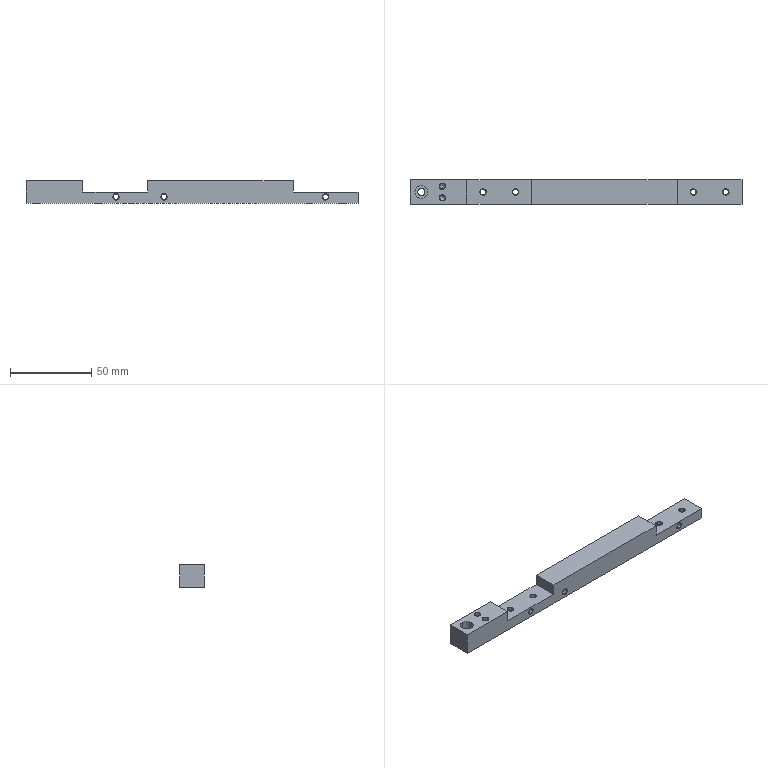CAM job | Mastercam | mm | 15 operations | part box 204.5 x 15 x 14
1. Facing | 24 - 100 平铣刀
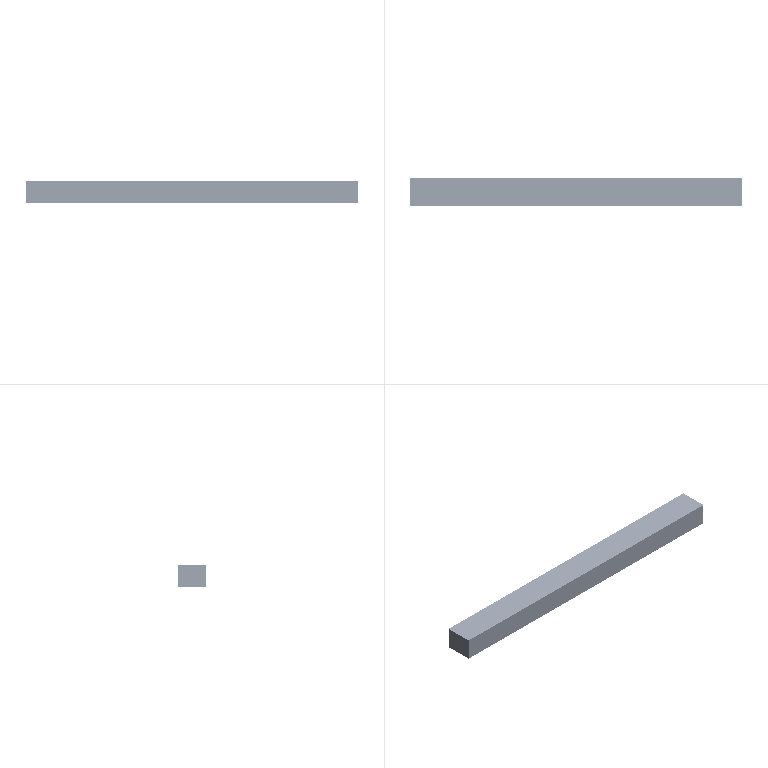2. Contour (Ramp) | 10 - 10 平铣刀
3. Contour (2D) | 8 - 8 平铣刀
4. Contour (2D chamfer) | 7 - 6 倒角刀
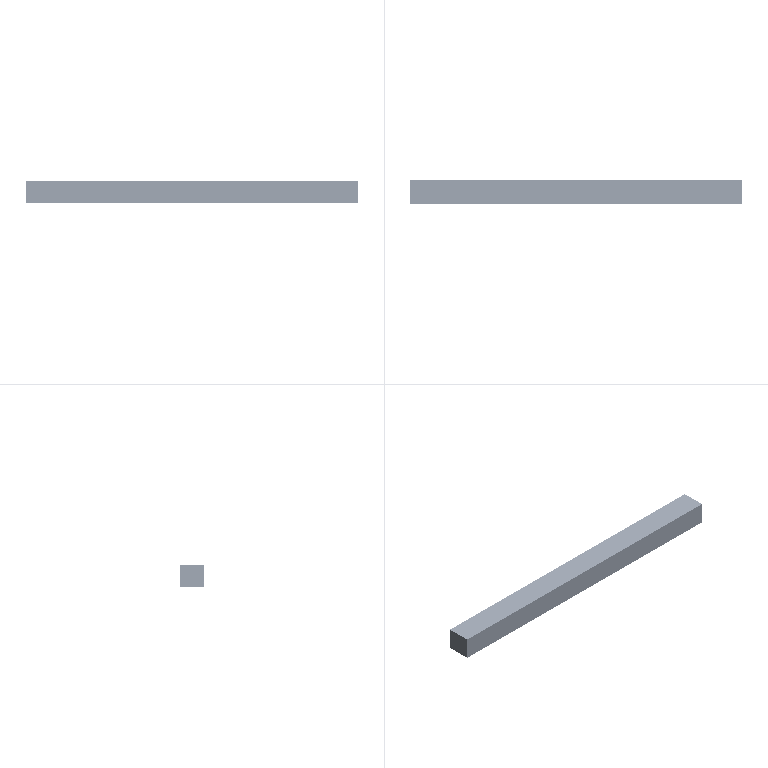5. Facing | 24 - 50 平铣刀
6. Contour (Ramp) | 10 - 10 平铣刀
7. Contour (2D) | 10 - 10 平铣刀
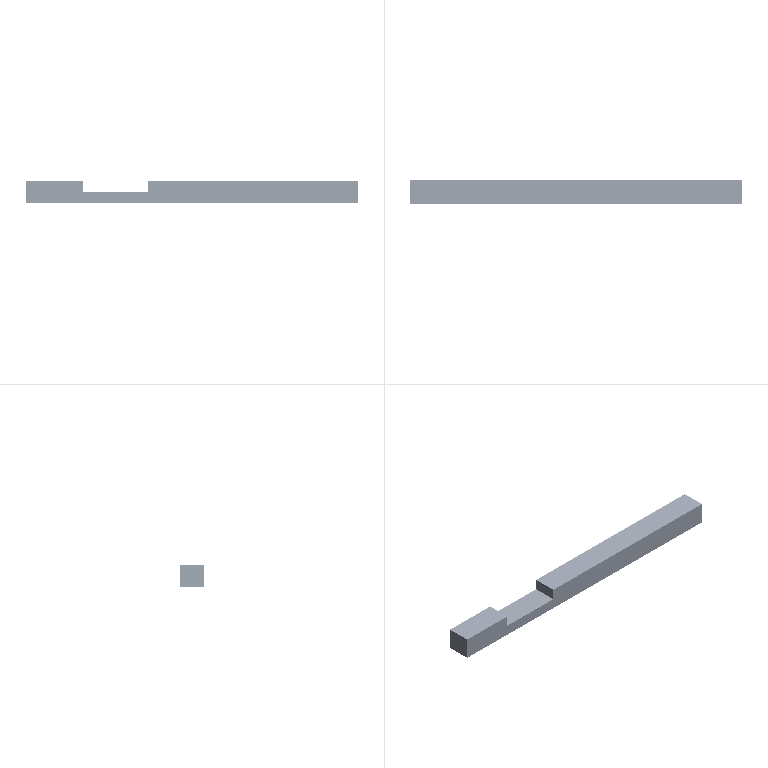8. Contour (Ramp) | 10 - 10 平铣刀
9. Contour (2D) | 10 - 10 平铣刀
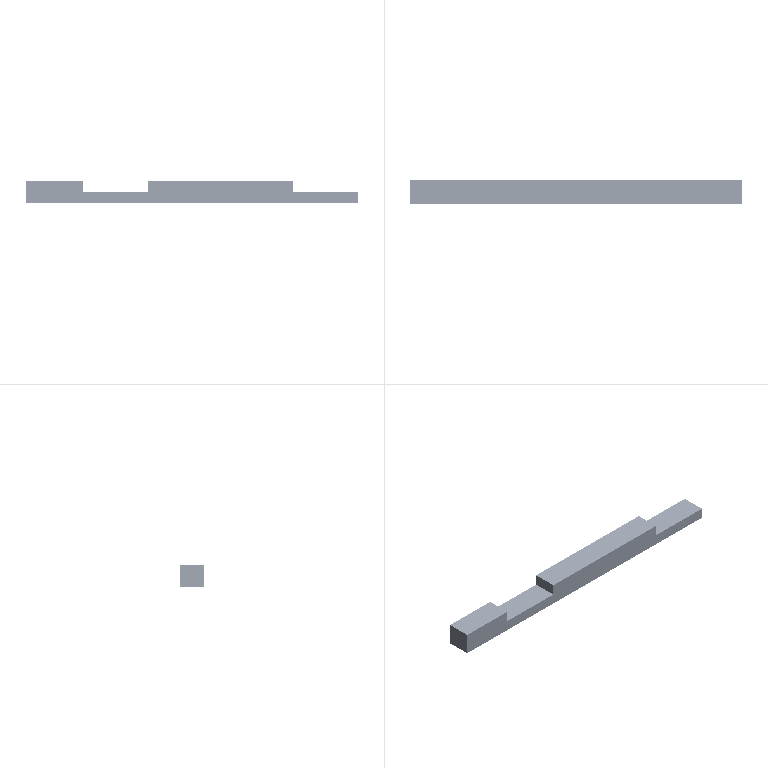10. Contour (Ramp) | 5 - 5 平铣刀
11. Contour (Ramp) | 5 - 5 平铣刀
12. Drill/Counterbore | 7 - 6 倒角刀
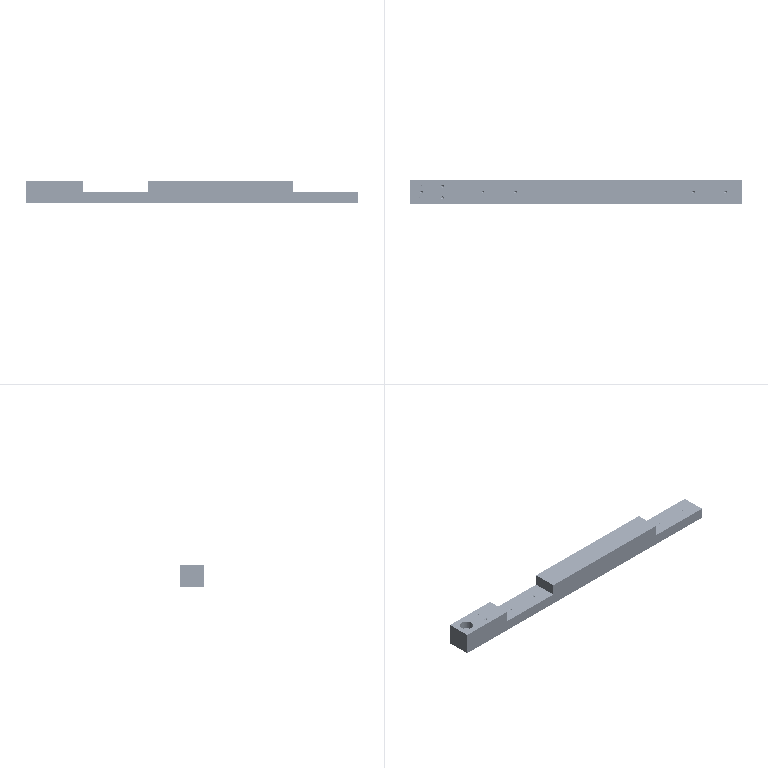13. Contour (2D chamfer) | 7 - 6 倒角刀
14. Contour (2D chamfer) | 7 - 6 倒角刀
15. Drill/Counterbore | 7 - 6 倒角刀